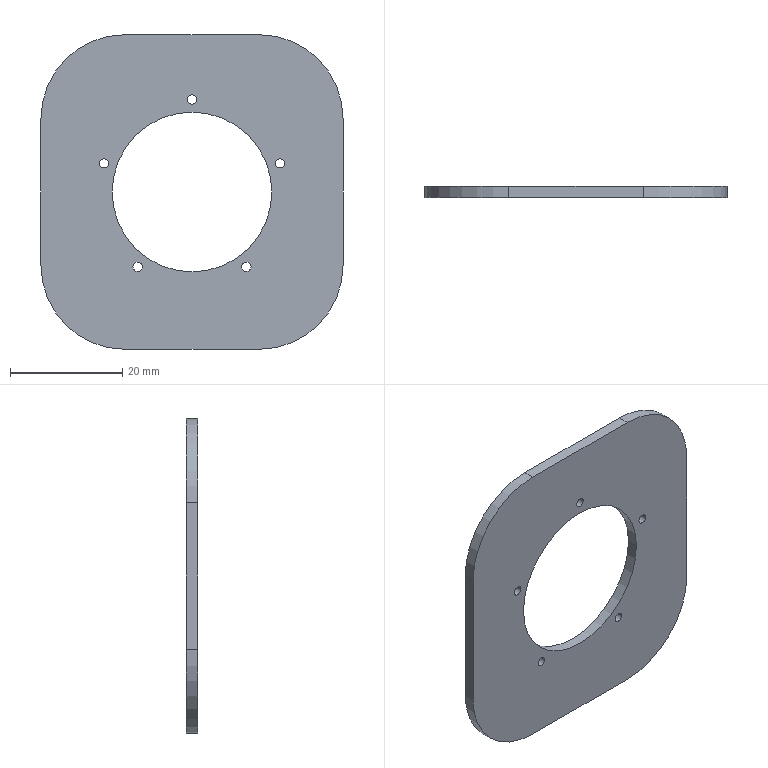Component | SolidWorks | BeanStorageBoxLid-1 | 1 solid | 22 faces | box 53.95 x 2 x 56.16 mm | volume 4376 mm3 | cylinder 16 | plane 6 | commonest cylinder face diameters 1.647 x10 30 x4 28.5 x2
build123d program:
from build123d import *

# Parameters (mm, degrees)
BOSS_EXTRUDE1_DEPTH = 2
SKETCH2_R           = 14.25
CUT_EXTRUDE1_DEPTH  = 2
SKETCH3_R           = 0.8233
CUT_EXTRUDE2_DEPTH  = 2
CIRPATTERN1_COUNT   = 5


with BuildPart() as part:
    # Sketch1 → Boss-Extrude1 (new body)
    with BuildSketch(Plane.XY):
        with BuildLine():
            Line((-11.975, -28.08), (11.975, -28.08))
            ThreePointArc((11.975, -28.08), (22.582, -23.687), (26.975, -13.08))
            Line((26.975, -13.08), (26.975, 13.08))
            ThreePointArc((26.975, 13.08), (22.582, 23.687), (11.975, 28.08))
            Line((11.975, 28.08), (-11.975, 28.08))
            ThreePointArc((-11.975, 28.08), (-22.582, 23.687), (-26.975, 13.08))
            Line((-26.975, 13.08), (-26.975, -13.08))
            ThreePointArc((-26.975, -13.08), (-22.582, -23.687), (-11.975, -28.08))
        make_face()
    extrude(amount=BOSS_EXTRUDE1_DEPTH)

    # Sketch2 → Cut-Extrude1 (cut)
    with BuildSketch(Plane.XY.offset(2)):
        Circle(SKETCH2_R)
    extrude(amount=-CUT_EXTRUDE1_DEPTH, mode=Mode.SUBTRACT)

    # Sketch3 → Cut-Extrude2 (cut)
    with BuildSketch(Plane.XY.offset(2)):
        with Locations((0, 16.523)):
            Circle(SKETCH3_R)
    cut_extrude2 = extrude(amount=-CUT_EXTRUDE2_DEPTH, mode=Mode.SUBTRACT)

    # CirPattern1: Cut-Extrude2 ×5 about axis
    cirpattern1_axis = Axis((0, 0, 0), (0, 0, 1))
    for i in range(1, CIRPATTERN1_COUNT):
        add(cut_extrude2.rotate(cirpattern1_axis, i * 360 / CIRPATTERN1_COUNT), mode=Mode.SUBTRACT)


solid = part.part

# Placed as in the assembly
solid = solid.moved(Location((-76.689, 22.584, 229.26), (90, 0, 0)))
STEP:
#1=COLOUR_RGB('',0.7922,0.8196,0.9333);
#2=FILL_AREA_STYLE_COLOUR('',#1);
#3=FILL_AREA_STYLE('',(#2));
#4=SURFACE_STYLE_FILL_AREA(#3);
#5=SURFACE_SIDE_STYLE('',(#4));
#6=SURFACE_STYLE_USAGE(.BOTH.,#5);
#7=PRESENTATION_STYLE_ASSIGNMENT((#6));
#8=CARTESIAN_POINT('',(-2.368,0.8104,9.227));
#9=VERTEX_POINT('',#8);
#10=CARTESIAN_POINT('',(-2.433,0.8104,9.227));
#11=VERTEX_POINT('',#10);
#12=CARTESIAN_POINT('',(-2.401,0.8104,9.227));
#13=DIRECTION('',(0.,1.,-0.));
#14=DIRECTION('',(-0.309,0.,0.9511));
#15=AXIS2_PLACEMENT_3D('',#12,#13,#14);
#16=CIRCLE('',#15,0.03241);
#17=EDGE_CURVE('',#9,#11,#16,.T.);
#18=ORIENTED_EDGE('',*,*,#17,.F.);
#19=CARTESIAN_POINT('',(-2.368,0.8891,9.227));
#20=VERTEX_POINT('',#19);
#21=CARTESIAN_POINT('',(-2.368,0.8104,9.227));
#22=DIRECTION('',(0.,1.,-0.));
#23=VECTOR('',#22,39.37);
#24=LINE('',#21,#23);
#25=EDGE_CURVE('',#9,#20,#24,.T.);
#26=ORIENTED_EDGE('',*,*,#25,.T.);
#27=CARTESIAN_POINT('',(-2.433,0.8891,9.227));
#28=VERTEX_POINT('',#27);
#29=CARTESIAN_POINT('',(-2.401,0.8891,9.227));
#30=DIRECTION('',(0.,1.,-0.));
#31=DIRECTION('',(-0.309,0.,0.9511));
#32=AXIS2_PLACEMENT_3D('',#29,#30,#31);
#33=CIRCLE('',#32,0.03241);
#34=EDGE_CURVE('',#20,#28,#33,.T.);
#35=ORIENTED_EDGE('',*,*,#34,.T.);
#36=CARTESIAN_POINT('',(-2.433,0.8104,9.227));
#37=DIRECTION('',(0.,1.,-0.));
#38=VECTOR('',#37,39.37);
#39=LINE('',#36,#38);
#40=EDGE_CURVE('',#11,#28,#39,.T.);
#41=ORIENTED_EDGE('',*,*,#40,.F.);
#42=EDGE_LOOP('',(#18,#26,#35,#41));
#43=FACE_OUTER_BOUND('',#42,.T.);
#44=CARTESIAN_POINT('',(-2.401,0.8104,9.227));
#45=DIRECTION('',(0.,1.,-0.));
#46=DIRECTION('',(-1.,0.,0.));
#47=AXIS2_PLACEMENT_3D('',#44,#45,#46);
#48=CYLINDRICAL_SURFACE('',#47,0.03241);
#49=ADVANCED_FACE('',(#43),#48,.F.);
#50=CARTESIAN_POINT('',(-2.604,0.8104,8.5));
#51=VERTEX_POINT('',#50);
#52=CARTESIAN_POINT('',(-2.669,0.8104,8.5));
#53=VERTEX_POINT('',#52);
#54=CARTESIAN_POINT('',(-2.637,0.8104,8.5));
#55=DIRECTION('',(0.,1.,-0.));
#56=DIRECTION('',(0.809,0.,0.5878));
#57=AXIS2_PLACEMENT_3D('',#54,#55,#56);
#58=CIRCLE('',#57,0.03241);
#59=EDGE_CURVE('',#51,#53,#58,.T.);
#60=ORIENTED_EDGE('',*,*,#59,.F.);
#61=CARTESIAN_POINT('',(-2.604,0.8891,8.5));
#62=VERTEX_POINT('',#61);
#63=CARTESIAN_POINT('',(-2.604,0.8104,8.5));
#64=DIRECTION('',(0.,1.,-0.));
#65=VECTOR('',#64,39.37);
#66=LINE('',#63,#65);
#67=EDGE_CURVE('',#51,#62,#66,.T.);
#68=ORIENTED_EDGE('',*,*,#67,.T.);
#69=CARTESIAN_POINT('',(-2.669,0.8891,8.5));
#70=VERTEX_POINT('',#69);
#71=CARTESIAN_POINT('',(-2.637,0.8891,8.5));
#72=DIRECTION('',(0.,1.,-0.));
#73=DIRECTION('',(0.809,0.,0.5878));
#74=AXIS2_PLACEMENT_3D('',#71,#72,#73);
#75=CIRCLE('',#74,0.03241);
#76=EDGE_CURVE('',#62,#70,#75,.T.);
#77=ORIENTED_EDGE('',*,*,#76,.T.);
#78=CARTESIAN_POINT('',(-2.669,0.8104,8.5));
#79=DIRECTION('',(0.,1.,-0.));
#80=VECTOR('',#79,39.37);
#81=LINE('',#78,#80);
#82=EDGE_CURVE('',#53,#70,#81,.T.);
#83=ORIENTED_EDGE('',*,*,#82,.F.);
#84=EDGE_LOOP('',(#60,#68,#77,#83));
#85=FACE_OUTER_BOUND('',#84,.T.);
#86=CARTESIAN_POINT('',(-2.637,0.8104,8.5));
#87=DIRECTION('',(0.,1.,-0.));
#88=DIRECTION('',(-1.,0.,0.));
#89=AXIS2_PLACEMENT_3D('',#86,#87,#88);
#90=CYLINDRICAL_SURFACE('',#89,0.03241);
#91=ADVANCED_FACE('',(#85),#90,.F.);
#92=CARTESIAN_POINT('',(-3.369,0.8104,8.5));
#93=VERTEX_POINT('',#92);
#94=CARTESIAN_POINT('',(-3.434,0.8104,8.5));
#95=VERTEX_POINT('',#94);
#96=CARTESIAN_POINT('',(-3.402,0.8104,8.5));
#97=DIRECTION('',(0.,1.,-0.));
#98=DIRECTION('',(0.809,0.,-0.5878));
#99=AXIS2_PLACEMENT_3D('',#96,#97,#98);
#100=CIRCLE('',#99,0.03241);
#101=EDGE_CURVE('',#93,#95,#100,.T.);
#102=ORIENTED_EDGE('',*,*,#101,.F.);
#103=CARTESIAN_POINT('',(-3.369,0.8891,8.5));
#104=VERTEX_POINT('',#103);
#105=CARTESIAN_POINT('',(-3.369,0.8104,8.5));
#106=DIRECTION('',(0.,1.,-0.));
#107=VECTOR('',#106,39.37);
#108=LINE('',#105,#107);
#109=EDGE_CURVE('',#93,#104,#108,.T.);
#110=ORIENTED_EDGE('',*,*,#109,.T.);
#111=CARTESIAN_POINT('',(-3.434,0.8891,8.5));
#112=VERTEX_POINT('',#111);
#113=CARTESIAN_POINT('',(-3.402,0.8891,8.5));
#114=DIRECTION('',(0.,1.,-0.));
#115=DIRECTION('',(0.809,0.,-0.5878));
#116=AXIS2_PLACEMENT_3D('',#113,#114,#115);
#117=CIRCLE('',#116,0.03241);
#118=EDGE_CURVE('',#104,#112,#117,.T.);
#119=ORIENTED_EDGE('',*,*,#118,.T.);
#120=CARTESIAN_POINT('',(-3.434,0.8104,8.5));
#121=DIRECTION('',(0.,1.,-0.));
#122=VECTOR('',#121,39.37);
#123=LINE('',#120,#122);
#124=EDGE_CURVE('',#95,#112,#123,.T.);
#125=ORIENTED_EDGE('',*,*,#124,.F.);
#126=EDGE_LOOP('',(#102,#110,#119,#125));
#127=FACE_OUTER_BOUND('',#126,.T.);
#128=CARTESIAN_POINT('',(-3.402,0.8104,8.5));
#129=DIRECTION('',(0.,1.,-0.));
#130=DIRECTION('',(-1.,0.,0.));
#131=AXIS2_PLACEMENT_3D('',#128,#129,#130);
#132=CYLINDRICAL_SURFACE('',#131,0.03241);
#133=ADVANCED_FACE('',(#127),#132,.F.);
#134=CARTESIAN_POINT('',(-3.606,0.8104,9.227));
#135=VERTEX_POINT('',#134);
#136=CARTESIAN_POINT('',(-3.67,0.8104,9.227));
#137=VERTEX_POINT('',#136);
#138=CARTESIAN_POINT('',(-3.638,0.8104,9.227));
#139=DIRECTION('',(0.,1.,-0.));
#140=DIRECTION('',(-0.309,0.,-0.9511));
#141=AXIS2_PLACEMENT_3D('',#138,#139,#140);
#142=CIRCLE('',#141,0.03241);
#143=EDGE_CURVE('',#135,#137,#142,.T.);
#144=ORIENTED_EDGE('',*,*,#143,.F.);
#145=CARTESIAN_POINT('',(-3.606,0.8891,9.227));
#146=VERTEX_POINT('',#145);
#147=CARTESIAN_POINT('',(-3.606,0.8104,9.227));
#148=DIRECTION('',(0.,1.,-0.));
#149=VECTOR('',#148,39.37);
#150=LINE('',#147,#149);
#151=EDGE_CURVE('',#135,#146,#150,.T.);
#152=ORIENTED_EDGE('',*,*,#151,.T.);
#153=CARTESIAN_POINT('',(-3.67,0.8891,9.227));
#154=VERTEX_POINT('',#153);
#155=CARTESIAN_POINT('',(-3.638,0.8891,9.227));
#156=DIRECTION('',(0.,1.,-0.));
#157=DIRECTION('',(-0.309,0.,-0.9511));
#158=AXIS2_PLACEMENT_3D('',#155,#156,#157);
#159=CIRCLE('',#158,0.03241);
#160=EDGE_CURVE('',#146,#154,#159,.T.);
#161=ORIENTED_EDGE('',*,*,#160,.T.);
#162=CARTESIAN_POINT('',(-3.67,0.8104,9.227));
#163=DIRECTION('',(0.,1.,-0.));
#164=VECTOR('',#163,39.37);
#165=LINE('',#162,#164);
#166=EDGE_CURVE('',#137,#154,#165,.T.);
#167=ORIENTED_EDGE('',*,*,#166,.F.);
#168=EDGE_LOOP('',(#144,#152,#161,#167));
#169=FACE_OUTER_BOUND('',#168,.T.);
#170=CARTESIAN_POINT('',(-3.638,0.8104,9.227));
#171=DIRECTION('',(0.,1.,-0.));
#172=DIRECTION('',(-1.,0.,0.));
#173=AXIS2_PLACEMENT_3D('',#170,#171,#172);
#174=CYLINDRICAL_SURFACE('',#173,0.03241);
#175=ADVANCED_FACE('',(#169),#174,.F.);
#176=CARTESIAN_POINT('',(-2.987,0.8104,9.676));
#177=VERTEX_POINT('',#176);
#178=CARTESIAN_POINT('',(-3.052,0.8104,9.676));
#179=VERTEX_POINT('',#178);
#180=CARTESIAN_POINT('',(-3.019,0.8104,9.676));
#181=DIRECTION('',(0.,1.,-0.));
#182=DIRECTION('',(-1.,0.,0.));
#183=AXIS2_PLACEMENT_3D('',#180,#181,#182);
#184=CIRCLE('',#183,0.03241);
#185=EDGE_CURVE('',#177,#179,#184,.T.);
#186=ORIENTED_EDGE('',*,*,#185,.F.);
#187=CARTESIAN_POINT('',(-2.987,0.8891,9.676));
#188=VERTEX_POINT('',#187);
#189=CARTESIAN_POINT('',(-2.987,0.8104,9.676));
#190=DIRECTION('',(0.,1.,-0.));
#191=VECTOR('',#190,39.37);
#192=LINE('',#189,#191);
#193=EDGE_CURVE('',#177,#188,#192,.T.);
#194=ORIENTED_EDGE('',*,*,#193,.T.);
#195=CARTESIAN_POINT('',(-3.052,0.8891,9.676));
#196=VERTEX_POINT('',#195);
#197=CARTESIAN_POINT('',(-3.019,0.8891,9.676));
#198=DIRECTION('',(0.,1.,-0.));
#199=DIRECTION('',(-1.,0.,0.));
#200=AXIS2_PLACEMENT_3D('',#197,#198,#199);
#201=CIRCLE('',#200,0.03241);
#202=EDGE_CURVE('',#188,#196,#201,.T.);
#203=ORIENTED_EDGE('',*,*,#202,.T.);
#204=CARTESIAN_POINT('',(-3.052,0.8104,9.676));
#205=DIRECTION('',(0.,1.,-0.));
#206=VECTOR('',#205,39.37);
#207=LINE('',#204,#206);
#208=EDGE_CURVE('',#179,#196,#207,.T.);
#209=ORIENTED_EDGE('',*,*,#208,.F.);
#210=EDGE_LOOP('',(#186,#194,#203,#209));
#211=FACE_OUTER_BOUND('',#210,.T.);
#212=CARTESIAN_POINT('',(-3.019,0.8104,9.676));
#213=DIRECTION('',(0.,1.,-0.));
#214=DIRECTION('',(-1.,0.,0.));
#215=AXIS2_PLACEMENT_3D('',#212,#213,#214);
#216=CYLINDRICAL_SURFACE('',#215,0.03241);
#217=ADVANCED_FACE('',(#211),#216,.F.);
#218=CARTESIAN_POINT('',(-2.458,0.8104,9.026));
#219=VERTEX_POINT('',#218);
#220=CARTESIAN_POINT('',(-3.58,0.8104,9.026));
#221=VERTEX_POINT('',#220);
#222=CARTESIAN_POINT('',(-3.019,0.8104,9.026));
#223=DIRECTION('',(0.,1.,-0.));
#224=DIRECTION('',(-1.,0.,0.));
#225=AXIS2_PLACEMENT_3D('',#222,#223,#224);
#226=CIRCLE('',#225,0.561);
#227=EDGE_CURVE('',#219,#221,#226,.T.);
#228=ORIENTED_EDGE('',*,*,#227,.F.);
#229=CARTESIAN_POINT('',(-2.458,0.8891,9.026));
#230=VERTEX_POINT('',#229);
#231=CARTESIAN_POINT('',(-2.458,0.8104,9.026));
#232=DIRECTION('',(0.,1.,-0.));
#233=VECTOR('',#232,39.37);
#234=LINE('',#231,#233);
#235=EDGE_CURVE('',#219,#230,#234,.T.);
#236=ORIENTED_EDGE('',*,*,#235,.T.);
#237=CARTESIAN_POINT('',(-3.58,0.8891,9.026));
#238=VERTEX_POINT('',#237);
#239=CARTESIAN_POINT('',(-3.019,0.8891,9.026));
#240=DIRECTION('',(0.,1.,-0.));
#241=DIRECTION('',(-1.,0.,0.));
#242=AXIS2_PLACEMENT_3D('',#239,#240,#241);
#243=CIRCLE('',#242,0.561);
#244=EDGE_CURVE('',#230,#238,#243,.T.);
#245=ORIENTED_EDGE('',*,*,#244,.T.);
#246=CARTESIAN_POINT('',(-3.58,0.8104,9.026));
#247=DIRECTION('',(0.,1.,-0.));
#248=VECTOR('',#247,39.37);
#249=LINE('',#246,#248);
#250=EDGE_CURVE('',#221,#238,#249,.T.);
#251=ORIENTED_EDGE('',*,*,#250,.F.);
#252=EDGE_LOOP('',(#228,#236,#245,#251));
#253=FACE_OUTER_BOUND('',#252,.T.);
#254=CARTESIAN_POINT('',(-3.019,0.8104,9.026));
#255=DIRECTION('',(0.,1.,-0.));
#256=DIRECTION('',(-1.,0.,0.));
#257=AXIS2_PLACEMENT_3D('',#254,#255,#256);
#258=CYLINDRICAL_SURFACE('',#257,0.561);
#259=ADVANCED_FACE('',(#253),#258,.F.);
#260=CARTESIAN_POINT('',(-1.957,0.8104,8.511));
#261=VERTEX_POINT('',#260);
#262=CARTESIAN_POINT('',(-2.548,0.8104,7.92));
#263=VERTEX_POINT('',#262);
#264=CARTESIAN_POINT('',(-2.548,0.8104,8.511));
#265=DIRECTION('',(0.,1.,-0.));
#266=DIRECTION('',(1.,0.,0.));
#267=AXIS2_PLACEMENT_3D('',#264,#265,#266);
#268=CIRCLE('',#267,0.5906);
#269=EDGE_CURVE('',#261,#263,#268,.T.);
#270=ORIENTED_EDGE('',*,*,#269,.T.);
#271=CARTESIAN_POINT('',(-2.548,0.8891,7.92));
#272=VERTEX_POINT('',#271);
#273=CARTESIAN_POINT('',(-2.548,0.8891,7.92));
#274=DIRECTION('',(-0.,-1.,0.));
#275=VECTOR('',#274,39.37);
#276=LINE('',#273,#275);
#277=EDGE_CURVE('',#272,#263,#276,.T.);
#278=ORIENTED_EDGE('',*,*,#277,.F.);
#279=CARTESIAN_POINT('',(-1.957,0.8891,8.511));
#280=VERTEX_POINT('',#279);
#281=CARTESIAN_POINT('',(-2.548,0.8891,8.511));
#282=DIRECTION('',(0.,1.,-0.));
#283=DIRECTION('',(1.,0.,0.));
#284=AXIS2_PLACEMENT_3D('',#281,#282,#283);
#285=CIRCLE('',#284,0.5906);
#286=EDGE_CURVE('',#280,#272,#285,.T.);
#287=ORIENTED_EDGE('',*,*,#286,.F.);
#288=CARTESIAN_POINT('',(-1.957,0.8891,8.511));
#289=DIRECTION('',(-0.,-1.,0.));
#290=VECTOR('',#289,39.37);
#291=LINE('',#288,#290);
#292=EDGE_CURVE('',#280,#261,#291,.T.);
#293=ORIENTED_EDGE('',*,*,#292,.T.);
#294=EDGE_LOOP('',(#270,#278,#287,#293));
#295=FACE_OUTER_BOUND('',#294,.T.);
#296=CARTESIAN_POINT('',(-2.548,0.8891,8.511));
#297=DIRECTION('',(-0.,-1.,0.));
#298=DIRECTION('',(1.,0.,0.));
#299=AXIS2_PLACEMENT_3D('',#296,#297,#298);
#300=CYLINDRICAL_SURFACE('',#299,0.5906);
#301=ADVANCED_FACE('',(#295),#300,.T.);
#302=CARTESIAN_POINT('',(-3.491,0.8104,7.92));
#303=VERTEX_POINT('',#302);
#304=CARTESIAN_POINT('',(-2.548,0.8104,7.92));
#305=DIRECTION('',(-1.,0.,0.));
#306=VECTOR('',#305,39.37);
#307=LINE('',#304,#306);
#308=EDGE_CURVE('',#263,#303,#307,.T.);
#309=ORIENTED_EDGE('',*,*,#308,.T.);
#310=CARTESIAN_POINT('',(-3.491,0.8891,7.92));
#311=VERTEX_POINT('',#310);
#312=CARTESIAN_POINT('',(-3.491,0.8891,7.92));
#313=DIRECTION('',(-0.,-1.,0.));
#314=VECTOR('',#313,39.37);
#315=LINE('',#312,#314);
#316=EDGE_CURVE('',#311,#303,#315,.T.);
#317=ORIENTED_EDGE('',*,*,#316,.F.);
#318=CARTESIAN_POINT('',(-2.548,0.8891,7.92));
#319=DIRECTION('',(-1.,0.,0.));
#320=VECTOR('',#319,39.37);
#321=LINE('',#318,#320);
#322=EDGE_CURVE('',#272,#311,#321,.T.);
#323=ORIENTED_EDGE('',*,*,#322,.F.);
#324=ORIENTED_EDGE('',*,*,#277,.T.);
#325=EDGE_LOOP('',(#309,#317,#323,#324));
#326=FACE_OUTER_BOUND('',#325,.T.);
#327=CARTESIAN_POINT('',(-2.548,0.8891,7.92));
#328=DIRECTION('',(0.,0.,1.));
#329=DIRECTION('',(0.,1.,-0.));
#330=AXIS2_PLACEMENT_3D('',#327,#328,#329);
#331=PLANE('',#330);
#332=ADVANCED_FACE('',(#326),#331,.F.);
#333=CARTESIAN_POINT('',(-4.081,0.8104,8.511));
#334=VERTEX_POINT('',#333);
#335=CARTESIAN_POINT('',(-3.491,0.8104,8.511));
#336=DIRECTION('',(0.,1.,-0.));
#337=DIRECTION('',(-1.,0.,0.));
#338=AXIS2_PLACEMENT_3D('',#335,#336,#337);
#339=CIRCLE('',#338,0.5906);
#340=EDGE_CURVE('',#303,#334,#339,.T.);
#341=ORIENTED_EDGE('',*,*,#340,.T.);
#342=CARTESIAN_POINT('',(-4.081,0.8891,8.511));
#343=VERTEX_POINT('',#342);
#344=CARTESIAN_POINT('',(-4.081,0.8891,8.511));
#345=DIRECTION('',(-0.,-1.,0.));
#346=VECTOR('',#345,39.37);
#347=LINE('',#344,#346);
#348=EDGE_CURVE('',#343,#334,#347,.T.);
#349=ORIENTED_EDGE('',*,*,#348,.F.);
#350=CARTESIAN_POINT('',(-3.491,0.8891,8.511));
#351=DIRECTION('',(0.,1.,-0.));
#352=DIRECTION('',(-1.,0.,0.));
#353=AXIS2_PLACEMENT_3D('',#350,#351,#352);
#354=CIRCLE('',#353,0.5906);
#355=EDGE_CURVE('',#311,#343,#354,.T.);
#356=ORIENTED_EDGE('',*,*,#355,.F.);
#357=ORIENTED_EDGE('',*,*,#316,.T.);
#358=EDGE_LOOP('',(#341,#349,#356,#357));
#359=FACE_OUTER_BOUND('',#358,.T.);
#360=CARTESIAN_POINT('',(-3.491,0.8891,8.511));
#361=DIRECTION('',(-0.,-1.,0.));
#362=DIRECTION('',(1.,0.,0.));
#363=AXIS2_PLACEMENT_3D('',#360,#361,#362);
#364=CYLINDRICAL_SURFACE('',#363,0.5906);
#365=ADVANCED_FACE('',(#359),#364,.T.);
#366=CARTESIAN_POINT('',(-4.081,0.8104,9.541));
#367=VERTEX_POINT('',#366);
#368=CARTESIAN_POINT('',(-4.081,0.8104,8.511));
#369=DIRECTION('',(0.,0.,1.));
#370=VECTOR('',#369,39.37);
#371=LINE('',#368,#370);
#372=EDGE_CURVE('',#334,#367,#371,.T.);
#373=ORIENTED_EDGE('',*,*,#372,.T.);
#374=CARTESIAN_POINT('',(-4.081,0.8891,9.541));
#375=VERTEX_POINT('',#374);
#376=CARTESIAN_POINT('',(-4.081,0.8891,9.541));
#377=DIRECTION('',(-0.,-1.,0.));
#378=VECTOR('',#377,39.37);
#379=LINE('',#376,#378);
#380=EDGE_CURVE('',#375,#367,#379,.T.);
#381=ORIENTED_EDGE('',*,*,#380,.F.);
#382=CARTESIAN_POINT('',(-4.081,0.8891,8.511));
#383=DIRECTION('',(0.,0.,1.));
#384=VECTOR('',#383,39.37);
#385=LINE('',#382,#384);
#386=EDGE_CURVE('',#343,#375,#385,.T.);
#387=ORIENTED_EDGE('',*,*,#386,.F.);
#388=ORIENTED_EDGE('',*,*,#348,.T.);
#389=EDGE_LOOP('',(#373,#381,#387,#388));
#390=FACE_OUTER_BOUND('',#389,.T.);
#391=CARTESIAN_POINT('',(-4.081,0.8891,8.511));
#392=DIRECTION('',(1.,-0.,-0.));
#393=DIRECTION('',(0.,1.,-0.));
#394=AXIS2_PLACEMENT_3D('',#391,#392,#393);
#395=PLANE('',#394);
#396=ADVANCED_FACE('',(#390),#395,.F.);
#397=CARTESIAN_POINT('',(-3.491,0.8104,10.131));
#398=VERTEX_POINT('',#397);
#399=CARTESIAN_POINT('',(-3.491,0.8104,9.541));
#400=DIRECTION('',(0.,1.,-0.));
#401=DIRECTION('',(1.,0.,0.));
#402=AXIS2_PLACEMENT_3D('',#399,#400,#401);
#403=CIRCLE('',#402,0.5906);
#404=EDGE_CURVE('',#367,#398,#403,.T.);
#405=ORIENTED_EDGE('',*,*,#404,.T.);
#406=CARTESIAN_POINT('',(-3.491,0.8891,10.131));
#407=VERTEX_POINT('',#406);
#408=CARTESIAN_POINT('',(-3.491,0.8891,10.131));
#409=DIRECTION('',(-0.,-1.,0.));
#410=VECTOR('',#409,39.37);
#411=LINE('',#408,#410);
#412=EDGE_CURVE('',#407,#398,#411,.T.);
#413=ORIENTED_EDGE('',*,*,#412,.F.);
#414=CARTESIAN_POINT('',(-3.491,0.8891,9.541));
#415=DIRECTION('',(0.,1.,-0.));
#416=DIRECTION('',(1.,0.,0.));
#417=AXIS2_PLACEMENT_3D('',#414,#415,#416);
#418=CIRCLE('',#417,0.5906);
#419=EDGE_CURVE('',#375,#407,#418,.T.);
#420=ORIENTED_EDGE('',*,*,#419,.F.);
#421=ORIENTED_EDGE('',*,*,#380,.T.);
#422=EDGE_LOOP('',(#405,#413,#420,#421));
#423=FACE_OUTER_BOUND('',#422,.T.);
#424=CARTESIAN_POINT('',(-3.491,0.8891,9.541));
#425=DIRECTION('',(-0.,-1.,0.));
#426=DIRECTION('',(1.,0.,0.));
#427=AXIS2_PLACEMENT_3D('',#424,#425,#426);
#428=CYLINDRICAL_SURFACE('',#427,0.5906);
#429=ADVANCED_FACE('',(#423),#428,.T.);
#430=CARTESIAN_POINT('',(-2.548,0.8104,10.131));
#431=VERTEX_POINT('',#430);
#432=CARTESIAN_POINT('',(-2.548,0.8104,10.131));
#433=DIRECTION('',(1.,-0.,-0.));
#434=VECTOR('',#433,39.37);
#435=LINE('',#432,#434);
#436=EDGE_CURVE('',#398,#431,#435,.T.);
#437=ORIENTED_EDGE('',*,*,#436,.T.);
#438=CARTESIAN_POINT('',(-2.548,0.8891,10.131));
#439=VERTEX_POINT('',#438);
#440=CARTESIAN_POINT('',(-2.548,0.8891,10.131));
#441=DIRECTION('',(-0.,-1.,0.));
#442=VECTOR('',#441,39.37);
#443=LINE('',#440,#442);
#444=EDGE_CURVE('',#439,#431,#443,.T.);
#445=ORIENTED_EDGE('',*,*,#444,.F.);
#446=CARTESIAN_POINT('',(-2.548,0.8891,10.131));
#447=DIRECTION('',(1.,-0.,-0.));
#448=VECTOR('',#447,39.37);
#449=LINE('',#446,#448);
#450=EDGE_CURVE('',#407,#439,#449,.T.);
#451=ORIENTED_EDGE('',*,*,#450,.F.);
#452=ORIENTED_EDGE('',*,*,#412,.T.);
#453=EDGE_LOOP('',(#437,#445,#451,#452));
#454=FACE_OUTER_BOUND('',#453,.T.);
#455=CARTESIAN_POINT('',(-2.548,0.8891,10.131));
#456=DIRECTION('',(-0.,-0.,-1.));
#457=DIRECTION('',(-0.,-1.,0.));
#458=AXIS2_PLACEMENT_3D('',#455,#456,#457);
#459=PLANE('',#458);
#460=ADVANCED_FACE('',(#454),#459,.F.);
#461=CARTESIAN_POINT('',(-1.957,0.8104,9.541));
#462=VERTEX_POINT('',#461);
#463=CARTESIAN_POINT('',(-2.548,0.8104,9.541));
#464=DIRECTION('',(0.,1.,-0.));
#465=DIRECTION('',(1.,0.,0.));
#466=AXIS2_PLACEMENT_3D('',#463,#464,#465);
#467=CIRCLE('',#466,0.5906);
#468=EDGE_CURVE('',#431,#462,#467,.T.);
#469=ORIENTED_EDGE('',*,*,#468,.T.);
#470=CARTESIAN_POINT('',(-1.957,0.8891,9.541));
#471=VERTEX_POINT('',#470);
#472=CARTESIAN_POINT('',(-1.957,0.8891,9.541));
#473=DIRECTION('',(-0.,-1.,0.));
#474=VECTOR('',#473,39.37);
#475=LINE('',#472,#474);
#476=EDGE_CURVE('',#471,#462,#475,.T.);
#477=ORIENTED_EDGE('',*,*,#476,.F.);
#478=CARTESIAN_POINT('',(-2.548,0.8891,9.541));
#479=DIRECTION('',(0.,1.,-0.));
#480=DIRECTION('',(1.,0.,0.));
#481=AXIS2_PLACEMENT_3D('',#478,#479,#480);
#482=CIRCLE('',#481,0.5906);
#483=EDGE_CURVE('',#439,#471,#482,.T.);
#484=ORIENTED_EDGE('',*,*,#483,.F.);
#485=ORIENTED_EDGE('',*,*,#444,.T.);
#486=EDGE_LOOP('',(#469,#477,#484,#485));
#487=FACE_OUTER_BOUND('',#486,.T.);
#488=CARTESIAN_POINT('',(-2.548,0.8891,9.541));
#489=DIRECTION('',(-0.,-1.,0.));
#490=DIRECTION('',(1.,0.,0.));
#491=AXIS2_PLACEMENT_3D('',#488,#489,#490);
#492=CYLINDRICAL_SURFACE('',#491,0.5906);
#493=ADVANCED_FACE('',(#487),#492,.T.);
#494=CARTESIAN_POINT('',(-1.957,0.8104,8.511));
#495=DIRECTION('',(-0.,-0.,-1.));
#496=VECTOR('',#495,39.37);
#497=LINE('',#494,#496);
#498=EDGE_CURVE('',#462,#261,#497,.T.);
#499=ORIENTED_EDGE('',*,*,#498,.T.);
#500=ORIENTED_EDGE('',*,*,#292,.F.);
#501=CARTESIAN_POINT('',(-1.957,0.8891,8.511));
#502=DIRECTION('',(-0.,-0.,-1.));
#503=VECTOR('',#502,39.37);
#504=LINE('',#501,#503);
#505=EDGE_CURVE('',#471,#280,#504,.T.);
#506=ORIENTED_EDGE('',*,*,#505,.F.);
#507=ORIENTED_EDGE('',*,*,#476,.T.);
#508=EDGE_LOOP('',(#499,#500,#506,#507));
#509=FACE_OUTER_BOUND('',#508,.T.);
#510=CARTESIAN_POINT('',(-1.957,0.8891,8.511));
#511=DIRECTION('',(-1.,0.,0.));
#512=DIRECTION('',(-0.,-1.,0.));
#513=AXIS2_PLACEMENT_3D('',#510,#511,#512);
#514=PLANE('',#513);
#515=ADVANCED_FACE('',(#509),#514,.F.);
#516=CARTESIAN_POINT('',(-2.401,0.8891,9.227));
#517=DIRECTION('',(0.,1.,-0.));
#518=DIRECTION('',(-0.309,0.,0.9511));
#519=AXIS2_PLACEMENT_3D('',#516,#517,#518);
#520=CIRCLE('',#519,0.03241);
#521=EDGE_CURVE('',#28,#20,#520,.T.);
#522=ORIENTED_EDGE('',*,*,#521,.F.);
#523=ORIENTED_EDGE('',*,*,#34,.F.);
#524=EDGE_LOOP('',(#522,#523));
#525=FACE_BOUND('',#524,.T.);
#526=CARTESIAN_POINT('',(-2.637,0.8891,8.5));
#527=DIRECTION('',(0.,1.,-0.));
#528=DIRECTION('',(0.809,0.,0.5878));
#529=AXIS2_PLACEMENT_3D('',#526,#527,#528);
#530=CIRCLE('',#529,0.03241);
#531=EDGE_CURVE('',#70,#62,#530,.T.);
#532=ORIENTED_EDGE('',*,*,#531,.F.);
#533=ORIENTED_EDGE('',*,*,#76,.F.);
#534=EDGE_LOOP('',(#532,#533));
#535=FACE_BOUND('',#534,.T.);
#536=CARTESIAN_POINT('',(-3.402,0.8891,8.5));
#537=DIRECTION('',(0.,1.,-0.));
#538=DIRECTION('',(0.809,0.,-0.5878));
#539=AXIS2_PLACEMENT_3D('',#536,#537,#538);
#540=CIRCLE('',#539,0.03241);
#541=EDGE_CURVE('',#112,#104,#540,.T.);
#542=ORIENTED_EDGE('',*,*,#541,.F.);
#543=ORIENTED_EDGE('',*,*,#118,.F.);
#544=EDGE_LOOP('',(#542,#543));
#545=FACE_BOUND('',#544,.T.);
#546=CARTESIAN_POINT('',(-3.638,0.8891,9.227));
#547=DIRECTION('',(0.,1.,-0.));
#548=DIRECTION('',(-0.309,0.,-0.9511));
#549=AXIS2_PLACEMENT_3D('',#546,#547,#548);
#550=CIRCLE('',#549,0.03241);
#551=EDGE_CURVE('',#154,#146,#550,.T.);
#552=ORIENTED_EDGE('',*,*,#551,.F.);
#553=ORIENTED_EDGE('',*,*,#160,.F.);
#554=EDGE_LOOP('',(#552,#553));
#555=FACE_BOUND('',#554,.T.);
#556=CARTESIAN_POINT('',(-3.019,0.8891,9.676));
#557=DIRECTION('',(0.,1.,-0.));
#558=DIRECTION('',(-1.,0.,0.));
#559=AXIS2_PLACEMENT_3D('',#556,#557,#558);
#560=CIRCLE('',#559,0.03241);
#561=EDGE_CURVE('',#196,#188,#560,.T.);
#562=ORIENTED_EDGE('',*,*,#561,.F.);
#563=ORIENTED_EDGE('',*,*,#202,.F.);
#564=EDGE_LOOP('',(#562,#563));
#565=FACE_BOUND('',#564,.T.);
#566=CARTESIAN_POINT('',(-3.019,0.8891,9.026));
#567=DIRECTION('',(0.,1.,-0.));
#568=DIRECTION('',(-1.,0.,0.));
#569=AXIS2_PLACEMENT_3D('',#566,#567,#568);
#570=CIRCLE('',#569,0.561);
#571=EDGE_CURVE('',#238,#230,#570,.T.);
#572=ORIENTED_EDGE('',*,*,#571,.F.);
#573=ORIENTED_EDGE('',*,*,#244,.F.);
#574=EDGE_LOOP('',(#572,#573));
#575=FACE_BOUND('',#574,.T.);
#576=ORIENTED_EDGE('',*,*,#286,.T.);
#577=ORIENTED_EDGE('',*,*,#322,.T.);
#578=ORIENTED_EDGE('',*,*,#355,.T.);
#579=ORIENTED_EDGE('',*,*,#386,.T.);
#580=ORIENTED_EDGE('',*,*,#419,.T.);
#581=ORIENTED_EDGE('',*,*,#450,.T.);
#582=ORIENTED_EDGE('',*,*,#483,.T.);
#583=ORIENTED_EDGE('',*,*,#505,.T.);
#584=EDGE_LOOP('',(#576,#577,#578,#579,#580,#581,#582,#583));
#585=FACE_OUTER_BOUND('',#584,.T.);
#586=CARTESIAN_POINT('',(-2.548,0.8891,8.511));
#587=DIRECTION('',(-0.,-1.,0.));
#588=DIRECTION('',(1.,-0.,-0.));
#589=AXIS2_PLACEMENT_3D('',#586,#587,#588);
#590=PLANE('',#589);
#591=ADVANCED_FACE('',(#525,#535,#545,#555,#565,#575,#585),#590,.F.);
#592=CARTESIAN_POINT('',(-2.401,0.8104,9.227));
#593=DIRECTION('',(0.,1.,-0.));
#594=DIRECTION('',(-0.309,0.,0.9511));
#595=AXIS2_PLACEMENT_3D('',#592,#593,#594);
#596=CIRCLE('',#595,0.03241);
#597=EDGE_CURVE('',#11,#9,#596,.T.);
#598=ORIENTED_EDGE('',*,*,#597,.T.);
#599=ORIENTED_EDGE('',*,*,#17,.T.);
#600=EDGE_LOOP('',(#598,#599));
#601=FACE_BOUND('',#600,.T.);
#602=CARTESIAN_POINT('',(-2.637,0.8104,8.5));
#603=DIRECTION('',(0.,1.,-0.));
#604=DIRECTION('',(0.809,0.,0.5878));
#605=AXIS2_PLACEMENT_3D('',#602,#603,#604);
#606=CIRCLE('',#605,0.03241);
#607=EDGE_CURVE('',#53,#51,#606,.T.);
#608=ORIENTED_EDGE('',*,*,#607,.T.);
#609=ORIENTED_EDGE('',*,*,#59,.T.);
#610=EDGE_LOOP('',(#608,#609));
#611=FACE_BOUND('',#610,.T.);
#612=CARTESIAN_POINT('',(-3.402,0.8104,8.5));
#613=DIRECTION('',(0.,1.,-0.));
#614=DIRECTION('',(0.809,0.,-0.5878));
#615=AXIS2_PLACEMENT_3D('',#612,#613,#614);
#616=CIRCLE('',#615,0.03241);
#617=EDGE_CURVE('',#95,#93,#616,.T.);
#618=ORIENTED_EDGE('',*,*,#617,.T.);
#619=ORIENTED_EDGE('',*,*,#101,.T.);
#620=EDGE_LOOP('',(#618,#619));
#621=FACE_BOUND('',#620,.T.);
#622=CARTESIAN_POINT('',(-3.638,0.8104,9.227));
#623=DIRECTION('',(0.,1.,-0.));
#624=DIRECTION('',(-0.309,0.,-0.9511));
#625=AXIS2_PLACEMENT_3D('',#622,#623,#624);
#626=CIRCLE('',#625,0.03241);
#627=EDGE_CURVE('',#137,#135,#626,.T.);
#628=ORIENTED_EDGE('',*,*,#627,.T.);
#629=ORIENTED_EDGE('',*,*,#143,.T.);
#630=EDGE_LOOP('',(#628,#629));
#631=FACE_BOUND('',#630,.T.);
#632=CARTESIAN_POINT('',(-3.019,0.8104,9.676));
#633=DIRECTION('',(0.,1.,-0.));
#634=DIRECTION('',(-1.,0.,0.));
#635=AXIS2_PLACEMENT_3D('',#632,#633,#634);
#636=CIRCLE('',#635,0.03241);
#637=EDGE_CURVE('',#179,#177,#636,.T.);
#638=ORIENTED_EDGE('',*,*,#637,.T.);
#639=ORIENTED_EDGE('',*,*,#185,.T.);
#640=EDGE_LOOP('',(#638,#639));
#641=FACE_BOUND('',#640,.T.);
#642=CARTESIAN_POINT('',(-3.019,0.8104,9.026));
#643=DIRECTION('',(0.,1.,-0.));
#644=DIRECTION('',(-1.,0.,0.));
#645=AXIS2_PLACEMENT_3D('',#642,#643,#644);
#646=CIRCLE('',#645,0.561);
#647=EDGE_CURVE('',#221,#219,#646,.T.);
#648=ORIENTED_EDGE('',*,*,#647,.T.);
#649=ORIENTED_EDGE('',*,*,#227,.T.);
#650=EDGE_LOOP('',(#648,#649));
#651=FACE_BOUND('',#650,.T.);
#652=ORIENTED_EDGE('',*,*,#269,.F.);
#653=ORIENTED_EDGE('',*,*,#498,.F.);
#654=ORIENTED_EDGE('',*,*,#468,.F.);
#655=ORIENTED_EDGE('',*,*,#436,.F.);
#656=ORIENTED_EDGE('',*,*,#404,.F.);
#657=ORIENTED_EDGE('',*,*,#372,.F.);
#658=ORIENTED_EDGE('',*,*,#340,.F.);
#659=ORIENTED_EDGE('',*,*,#308,.F.);
#660=EDGE_LOOP('',(#652,#653,#654,#655,#656,#657,#658,#659));
#661=FACE_OUTER_BOUND('',#660,.T.);
#662=CARTESIAN_POINT('',(-2.548,0.8104,8.511));
#663=DIRECTION('',(-0.,-1.,0.));
#664=DIRECTION('',(1.,-0.,-0.));
#665=AXIS2_PLACEMENT_3D('',#662,#663,#664);
#666=PLANE('',#665);
#667=ADVANCED_FACE('',(#601,#611,#621,#631,#641,#651,#661),#666,.T.);
#668=ORIENTED_EDGE('',*,*,#235,.F.);
#669=ORIENTED_EDGE('',*,*,#647,.F.);
#670=ORIENTED_EDGE('',*,*,#250,.T.);
#671=ORIENTED_EDGE('',*,*,#571,.T.);
#672=EDGE_LOOP('',(#668,#669,#670,#671));
#673=FACE_OUTER_BOUND('',#672,.T.);
#674=CARTESIAN_POINT('',(-3.019,0.8104,9.026));
#675=DIRECTION('',(0.,1.,-0.));
#676=DIRECTION('',(-1.,0.,0.));
#677=AXIS2_PLACEMENT_3D('',#674,#675,#676);
#678=CYLINDRICAL_SURFACE('',#677,0.561);
#679=ADVANCED_FACE('',(#673),#678,.F.);
#680=ORIENTED_EDGE('',*,*,#193,.F.);
#681=ORIENTED_EDGE('',*,*,#637,.F.);
#682=ORIENTED_EDGE('',*,*,#208,.T.);
#683=ORIENTED_EDGE('',*,*,#561,.T.);
#684=EDGE_LOOP('',(#680,#681,#682,#683));
#685=FACE_OUTER_BOUND('',#684,.T.);
#686=CARTESIAN_POINT('',(-3.019,0.8104,9.676));
#687=DIRECTION('',(0.,1.,-0.));
#688=DIRECTION('',(-1.,0.,0.));
#689=AXIS2_PLACEMENT_3D('',#686,#687,#688);
#690=CYLINDRICAL_SURFACE('',#689,0.03241);
#691=ADVANCED_FACE('',(#685),#690,.F.);
#692=ORIENTED_EDGE('',*,*,#151,.F.);
#693=ORIENTED_EDGE('',*,*,#627,.F.);
#694=ORIENTED_EDGE('',*,*,#166,.T.);
#695=ORIENTED_EDGE('',*,*,#551,.T.);
#696=EDGE_LOOP('',(#692,#693,#694,#695));
#697=FACE_OUTER_BOUND('',#696,.T.);
#698=CARTESIAN_POINT('',(-3.638,0.8104,9.227));
#699=DIRECTION('',(0.,1.,-0.));
#700=DIRECTION('',(-1.,0.,0.));
#701=AXIS2_PLACEMENT_3D('',#698,#699,#700);
#702=CYLINDRICAL_SURFACE('',#701,0.03241);
#703=ADVANCED_FACE('',(#697),#702,.F.);
#704=ORIENTED_EDGE('',*,*,#109,.F.);
#705=ORIENTED_EDGE('',*,*,#617,.F.);
#706=ORIENTED_EDGE('',*,*,#124,.T.);
#707=ORIENTED_EDGE('',*,*,#541,.T.);
#708=EDGE_LOOP('',(#704,#705,#706,#707));
#709=FACE_OUTER_BOUND('',#708,.T.);
#710=CARTESIAN_POINT('',(-3.402,0.8104,8.5));
#711=DIRECTION('',(0.,1.,-0.));
#712=DIRECTION('',(-1.,0.,0.));
#713=AXIS2_PLACEMENT_3D('',#710,#711,#712);
#714=CYLINDRICAL_SURFACE('',#713,0.03241);
#715=ADVANCED_FACE('',(#709),#714,.F.);
#716=ORIENTED_EDGE('',*,*,#67,.F.);
#717=ORIENTED_EDGE('',*,*,#607,.F.);
#718=ORIENTED_EDGE('',*,*,#82,.T.);
#719=ORIENTED_EDGE('',*,*,#531,.T.);
#720=EDGE_LOOP('',(#716,#717,#718,#719));
#721=FACE_OUTER_BOUND('',#720,.T.);
#722=CARTESIAN_POINT('',(-2.637,0.8104,8.5));
#723=DIRECTION('',(0.,1.,-0.));
#724=DIRECTION('',(-1.,0.,0.));
#725=AXIS2_PLACEMENT_3D('',#722,#723,#724);
#726=CYLINDRICAL_SURFACE('',#725,0.03241);
#727=ADVANCED_FACE('',(#721),#726,.F.);
#728=ORIENTED_EDGE('',*,*,#25,.F.);
#729=ORIENTED_EDGE('',*,*,#597,.F.);
#730=ORIENTED_EDGE('',*,*,#40,.T.);
#731=ORIENTED_EDGE('',*,*,#521,.T.);
#732=EDGE_LOOP('',(#728,#729,#730,#731));
#733=FACE_OUTER_BOUND('',#732,.T.);
#734=CARTESIAN_POINT('',(-2.401,0.8104,9.227));
#735=DIRECTION('',(0.,1.,-0.));
#736=DIRECTION('',(-1.,0.,0.));
#737=AXIS2_PLACEMENT_3D('',#734,#735,#736);
#738=CYLINDRICAL_SURFACE('',#737,0.03241);
#739=ADVANCED_FACE('',(#733),#738,.F.);
#740=CLOSED_SHELL('',(#49,#91,#133,#175,#217,#259,#301,#332,#365,#396,#429,#460,#493,#515,#591,#667,#679,#691,#703,#715,#727,#739));
#741=MANIFOLD_SOLID_BREP('',#740);
#742=STYLED_ITEM('',(#7),#741);
#743=PRESENTATION_LAYER_ASSIGNMENT('','',(#742));
#744=(LENGTH_UNIT()NAMED_UNIT(*)SI_UNIT($,.METRE.));
#745=LENGTH_MEASURE_WITH_UNIT(LENGTH_MEASURE(0.0254),#744);
#746=DIMENSIONAL_EXPONENTS(1.,0.,0.,0.,0.,0.,0.);
#747=(CONVERSION_BASED_UNIT('',#745)LENGTH_UNIT()NAMED_UNIT(#746));
#748=UNCERTAINTY_MEASURE_WITH_UNIT(LENGTH_MEASURE(0.00001),#747,'','');
#749=(NAMED_UNIT(*)PLANE_ANGLE_UNIT()SI_UNIT($,.RADIAN.));
#750=(NAMED_UNIT(*)SI_UNIT($,.STERADIAN.)SOLID_ANGLE_UNIT());
#751=(GEOMETRIC_REPRESENTATION_CONTEXT(3)GLOBAL_UNCERTAINTY_ASSIGNED_CONTEXT((#748))GLOBAL_UNIT_ASSIGNED_CONTEXT((#747,#749,#750))REPRESENTATION_CONTEXT('',''));
#752=MECHANICAL_DESIGN_GEOMETRIC_PRESENTATION_REPRESENTATION('',(#742),#751);
#753=CARTESIAN_POINT('',(0.,0.,0.));
#754=DIRECTION('',(0.,0.,1.));
#755=DIRECTION('',(1.,0.,0.));
#756=AXIS2_PLACEMENT_3D('',#753,#754,#755);
#757=(LENGTH_UNIT()NAMED_UNIT(*)SI_UNIT($,.METRE.));
#758=LENGTH_MEASURE_WITH_UNIT(LENGTH_MEASURE(0.0254),#757);
#759=DIMENSIONAL_EXPONENTS(1.,0.,0.,0.,0.,0.,0.);
#760=(CONVERSION_BASED_UNIT('',#758)LENGTH_UNIT()NAMED_UNIT(#759));
#761=UNCERTAINTY_MEASURE_WITH_UNIT(LENGTH_MEASURE(0.00001),#760,'','');
#762=(NAMED_UNIT(*)PLANE_ANGLE_UNIT()SI_UNIT($,.RADIAN.));
#763=(NAMED_UNIT(*)SI_UNIT($,.STERADIAN.)SOLID_ANGLE_UNIT());
#764=(GEOMETRIC_REPRESENTATION_CONTEXT(3)GLOBAL_UNCERTAINTY_ASSIGNED_CONTEXT((#761))GLOBAL_UNIT_ASSIGNED_CONTEXT((#760,#762,#763))REPRESENTATION_CONTEXT('',''));
#765=ADVANCED_BREP_SHAPE_REPRESENTATION('',(#741,#756),#764);